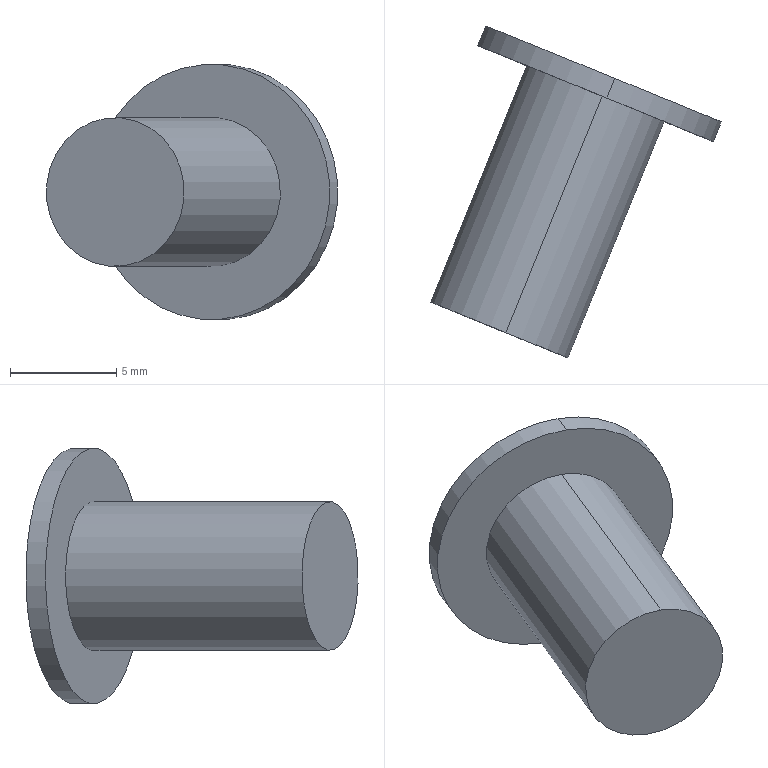Component | SolidWorks | FixedWingPin-11 | 1 solid | 7 faces | box 13.7 x 15.62 x 12 mm | volume 575 mm3 | cylinder 4 | plane 3 | commonest cylinder face diameters 12 x2 7 x2
build123d program:
from build123d import *

# Parameters (mm, degrees)
SKETCH1_R           = 3.5
BOSS_EXTRUDE1_DEPTH = 12
SKETCH2_R           = 6
BOSS_EXTRUDE2_DEPTH = 1


with BuildPart() as part:
    # Sketch1 → Boss-Extrude1 (new body)
    with BuildSketch(Plane.XY):
        with Locations((-274.486, -160)):
            Circle(SKETCH1_R)
    extrude(amount=-BOSS_EXTRUDE1_DEPTH)

    # Sketch2 → Boss-Extrude2 (add)
    with BuildSketch(Plane.XY):
        with Locations((-274.486, -160)):
            Circle(SKETCH2_R)
    extrude(amount=BOSS_EXTRUDE2_DEPTH)


solid = part.part

# Placed as in the assembly
solid = solid.moved(Location((-143.809, 26.687, -192.108), (-90, 22.15, 76.477)))
STEP:
#1=COLOUR_RGB('',0.7922,0.8196,0.9333);
#2=FILL_AREA_STYLE_COLOUR('',#1);
#3=FILL_AREA_STYLE('',(#2));
#4=SURFACE_STYLE_FILL_AREA(#3);
#5=SURFACE_SIDE_STYLE('',(#4));
#6=SURFACE_STYLE_USAGE(.BOTH.,#5);
#7=PRESENTATION_STYLE_ASSIGNMENT((#6));
#8=CARTESIAN_POINT('',(-2.336,-0.2608,4.181));
#9=VERTEX_POINT('',#8);
#10=CARTESIAN_POINT('',(-2.294,-0.2778,4.652));
#11=VERTEX_POINT('',#10);
#12=CARTESIAN_POINT('',(-2.315,-0.2693,4.417));
#13=DIRECTION('',(0.377,0.9262,0.));
#14=DIRECTION('',(-0.08843,0.036,-0.9954));
#15=AXIS2_PLACEMENT_3D('',#12,#13,#14);
#16=CIRCLE('',#15,0.2362);
#17=EDGE_CURVE('',#9,#11,#16,.T.);
#18=ORIENTED_EDGE('',*,*,#17,.F.);
#19=CARTESIAN_POINT('',(-2.351,-0.2972,4.181));
#20=VERTEX_POINT('',#19);
#21=CARTESIAN_POINT('',(-2.336,-0.2608,4.181));
#22=DIRECTION('',(-0.377,-0.9262,-0.));
#23=VECTOR('',#22,39.37);
#24=LINE('',#21,#23);
#25=EDGE_CURVE('',#9,#20,#24,.T.);
#26=ORIENTED_EDGE('',*,*,#25,.T.);
#27=CARTESIAN_POINT('',(-2.309,-0.3142,4.652));
#28=VERTEX_POINT('',#27);
#29=CARTESIAN_POINT('',(-2.33,-0.3057,4.417));
#30=DIRECTION('',(0.377,0.9262,0.));
#31=DIRECTION('',(-0.08843,0.036,-0.9954));
#32=AXIS2_PLACEMENT_3D('',#29,#30,#31);
#33=CIRCLE('',#32,0.2362);
#34=EDGE_CURVE('',#20,#28,#33,.T.);
#35=ORIENTED_EDGE('',*,*,#34,.T.);
#36=CARTESIAN_POINT('',(-2.294,-0.2778,4.652));
#37=DIRECTION('',(-0.377,-0.9262,-0.));
#38=VECTOR('',#37,39.37);
#39=LINE('',#36,#38);
#40=EDGE_CURVE('',#11,#28,#39,.T.);
#41=ORIENTED_EDGE('',*,*,#40,.F.);
#42=EDGE_LOOP('',(#18,#26,#35,#41));
#43=FACE_OUTER_BOUND('',#42,.T.);
#44=CARTESIAN_POINT('',(-2.315,-0.2693,4.417));
#45=DIRECTION('',(-0.377,-0.9262,-0.));
#46=DIRECTION('',(0.08843,-0.036,0.9954));
#47=AXIS2_PLACEMENT_3D('',#44,#45,#46);
#48=CYLINDRICAL_SURFACE('',#47,0.2362);
#49=ADVANCED_FACE('',(#43),#48,.T.);
#50=CARTESIAN_POINT('',(-2.52,-0.7384,4.279));
#51=VERTEX_POINT('',#50);
#52=CARTESIAN_POINT('',(-2.496,-0.7483,4.554));
#53=VERTEX_POINT('',#52);
#54=CARTESIAN_POINT('',(-2.508,-0.7433,4.417));
#55=DIRECTION('',(0.377,0.9262,0.));
#56=DIRECTION('',(-0.08843,0.036,-0.9954));
#57=AXIS2_PLACEMENT_3D('',#54,#55,#56);
#58=CIRCLE('',#57,0.1378);
#59=EDGE_CURVE('',#51,#53,#58,.T.);
#60=ORIENTED_EDGE('',*,*,#59,.T.);
#61=CARTESIAN_POINT('',(-2.318,-0.3107,4.554));
#62=VERTEX_POINT('',#61);
#63=CARTESIAN_POINT('',(-2.496,-0.7483,4.554));
#64=DIRECTION('',(0.377,0.9262,0.));
#65=VECTOR('',#64,39.37);
#66=LINE('',#63,#65);
#67=EDGE_CURVE('',#53,#62,#66,.T.);
#68=ORIENTED_EDGE('',*,*,#67,.T.);
#69=CARTESIAN_POINT('',(-2.342,-0.3008,4.279));
#70=VERTEX_POINT('',#69);
#71=CARTESIAN_POINT('',(-2.33,-0.3057,4.417));
#72=DIRECTION('',(0.377,0.9262,0.));
#73=DIRECTION('',(-0.08843,0.036,-0.9954));
#74=AXIS2_PLACEMENT_3D('',#71,#72,#73);
#75=CIRCLE('',#74,0.1378);
#76=EDGE_CURVE('',#70,#62,#75,.T.);
#77=ORIENTED_EDGE('',*,*,#76,.F.);
#78=CARTESIAN_POINT('',(-2.52,-0.7384,4.279));
#79=DIRECTION('',(0.377,0.9262,0.));
#80=VECTOR('',#79,39.37);
#81=LINE('',#78,#80);
#82=EDGE_CURVE('',#51,#70,#81,.T.);
#83=ORIENTED_EDGE('',*,*,#82,.F.);
#84=EDGE_LOOP('',(#60,#68,#77,#83));
#85=FACE_OUTER_BOUND('',#84,.T.);
#86=CARTESIAN_POINT('',(-2.508,-0.7433,4.417));
#87=DIRECTION('',(0.377,0.9262,0.));
#88=DIRECTION('',(-0.08843,0.036,-0.9954));
#89=AXIS2_PLACEMENT_3D('',#86,#87,#88);
#90=CYLINDRICAL_SURFACE('',#89,0.1378);
#91=ADVANCED_FACE('',(#85),#90,.T.);
#92=ORIENTED_EDGE('',*,*,#67,.F.);
#93=CARTESIAN_POINT('',(-2.508,-0.7433,4.417));
#94=DIRECTION('',(0.377,0.9262,0.));
#95=DIRECTION('',(-0.08843,0.036,-0.9954));
#96=AXIS2_PLACEMENT_3D('',#93,#94,#95);
#97=CIRCLE('',#96,0.1378);
#98=EDGE_CURVE('',#53,#51,#97,.T.);
#99=ORIENTED_EDGE('',*,*,#98,.T.);
#100=ORIENTED_EDGE('',*,*,#82,.T.);
#101=CARTESIAN_POINT('',(-2.33,-0.3057,4.417));
#102=DIRECTION('',(0.377,0.9262,0.));
#103=DIRECTION('',(-0.08843,0.036,-0.9954));
#104=AXIS2_PLACEMENT_3D('',#101,#102,#103);
#105=CIRCLE('',#104,0.1378);
#106=EDGE_CURVE('',#62,#70,#105,.T.);
#107=ORIENTED_EDGE('',*,*,#106,.F.);
#108=EDGE_LOOP('',(#92,#99,#100,#107));
#109=FACE_OUTER_BOUND('',#108,.T.);
#110=CARTESIAN_POINT('',(-2.508,-0.7433,4.417));
#111=DIRECTION('',(0.377,0.9262,0.));
#112=DIRECTION('',(-0.08843,0.036,-0.9954));
#113=AXIS2_PLACEMENT_3D('',#110,#111,#112);
#114=CYLINDRICAL_SURFACE('',#113,0.1378);
#115=ADVANCED_FACE('',(#109),#114,.T.);
#116=ORIENTED_EDGE('',*,*,#59,.F.);
#117=ORIENTED_EDGE('',*,*,#98,.F.);
#118=EDGE_LOOP('',(#116,#117));
#119=FACE_OUTER_BOUND('',#118,.T.);
#120=CARTESIAN_POINT('',(-2.508,-0.7433,4.417));
#121=DIRECTION('',(0.377,0.9262,0.));
#122=DIRECTION('',(-0.08843,0.036,-0.9954));
#123=AXIS2_PLACEMENT_3D('',#120,#121,#122);
#124=PLANE('',#123);
#125=ADVANCED_FACE('',(#119),#124,.F.);
#126=ORIENTED_EDGE('',*,*,#25,.F.);
#127=CARTESIAN_POINT('',(-2.315,-0.2693,4.417));
#128=DIRECTION('',(0.377,0.9262,0.));
#129=DIRECTION('',(-0.08843,0.036,-0.9954));
#130=AXIS2_PLACEMENT_3D('',#127,#128,#129);
#131=CIRCLE('',#130,0.2362);
#132=EDGE_CURVE('',#11,#9,#131,.T.);
#133=ORIENTED_EDGE('',*,*,#132,.F.);
#134=ORIENTED_EDGE('',*,*,#40,.T.);
#135=CARTESIAN_POINT('',(-2.33,-0.3057,4.417));
#136=DIRECTION('',(0.377,0.9262,0.));
#137=DIRECTION('',(-0.08843,0.036,-0.9954));
#138=AXIS2_PLACEMENT_3D('',#135,#136,#137);
#139=CIRCLE('',#138,0.2362);
#140=EDGE_CURVE('',#28,#20,#139,.T.);
#141=ORIENTED_EDGE('',*,*,#140,.T.);
#142=EDGE_LOOP('',(#126,#133,#134,#141));
#143=FACE_OUTER_BOUND('',#142,.T.);
#144=CARTESIAN_POINT('',(-2.315,-0.2693,4.417));
#145=DIRECTION('',(-0.377,-0.9262,-0.));
#146=DIRECTION('',(0.08843,-0.036,0.9954));
#147=AXIS2_PLACEMENT_3D('',#144,#145,#146);
#148=CYLINDRICAL_SURFACE('',#147,0.2362);
#149=ADVANCED_FACE('',(#143),#148,.T.);
#150=ORIENTED_EDGE('',*,*,#132,.T.);
#151=ORIENTED_EDGE('',*,*,#17,.T.);
#152=EDGE_LOOP('',(#150,#151));
#153=FACE_OUTER_BOUND('',#152,.T.);
#154=CARTESIAN_POINT('',(-2.315,-0.2693,4.417));
#155=DIRECTION('',(0.377,0.9262,0.));
#156=DIRECTION('',(-0.08843,0.036,-0.9954));
#157=AXIS2_PLACEMENT_3D('',#154,#155,#156);
#158=PLANE('',#157);
#159=ADVANCED_FACE('',(#153),#158,.T.);
#160=ORIENTED_EDGE('',*,*,#76,.T.);
#161=ORIENTED_EDGE('',*,*,#106,.T.);
#162=EDGE_LOOP('',(#160,#161));
#163=FACE_BOUND('',#162,.T.);
#164=ORIENTED_EDGE('',*,*,#140,.F.);
#165=ORIENTED_EDGE('',*,*,#34,.F.);
#166=EDGE_LOOP('',(#164,#165));
#167=FACE_OUTER_BOUND('',#166,.T.);
#168=CARTESIAN_POINT('',(-2.33,-0.3057,4.417));
#169=DIRECTION('',(0.377,0.9262,0.));
#170=DIRECTION('',(-0.08843,0.036,-0.9954));
#171=AXIS2_PLACEMENT_3D('',#168,#169,#170);
#172=PLANE('',#171);
#173=ADVANCED_FACE('',(#163,#167),#172,.F.);
#174=CLOSED_SHELL('',(#49,#91,#115,#125,#149,#159,#173));
#175=MANIFOLD_SOLID_BREP('',#174);
#176=STYLED_ITEM('',(#7),#175);
#177=(LENGTH_UNIT()NAMED_UNIT(*)SI_UNIT($,.METRE.));
#178=LENGTH_MEASURE_WITH_UNIT(LENGTH_MEASURE(0.0254),#177);
#179=DIMENSIONAL_EXPONENTS(1.,0.,0.,0.,0.,0.,0.);
#180=(CONVERSION_BASED_UNIT('',#178)LENGTH_UNIT()NAMED_UNIT(#179));
#181=UNCERTAINTY_MEASURE_WITH_UNIT(LENGTH_MEASURE(0.00001),#180,'','');
#182=(NAMED_UNIT(*)PLANE_ANGLE_UNIT()SI_UNIT($,.RADIAN.));
#183=(NAMED_UNIT(*)SI_UNIT($,.STERADIAN.)SOLID_ANGLE_UNIT());
#184=(GEOMETRIC_REPRESENTATION_CONTEXT(3)GLOBAL_UNCERTAINTY_ASSIGNED_CONTEXT((#181))GLOBAL_UNIT_ASSIGNED_CONTEXT((#180,#182,#183))REPRESENTATION_CONTEXT('',''));
#185=MECHANICAL_DESIGN_GEOMETRIC_PRESENTATION_REPRESENTATION('',(#176),#184);
#186=CARTESIAN_POINT('',(0.,0.,0.));
#187=DIRECTION('',(0.,0.,1.));
#188=DIRECTION('',(1.,0.,0.));
#189=AXIS2_PLACEMENT_3D('',#186,#187,#188);
#190=(LENGTH_UNIT()NAMED_UNIT(*)SI_UNIT($,.METRE.));
#191=LENGTH_MEASURE_WITH_UNIT(LENGTH_MEASURE(0.0254),#190);
#192=DIMENSIONAL_EXPONENTS(1.,0.,0.,0.,0.,0.,0.);
#193=(CONVERSION_BASED_UNIT('',#191)LENGTH_UNIT()NAMED_UNIT(#192));
#194=UNCERTAINTY_MEASURE_WITH_UNIT(LENGTH_MEASURE(0.00001),#193,'','');
#195=(NAMED_UNIT(*)PLANE_ANGLE_UNIT()SI_UNIT($,.RADIAN.));
#196=(NAMED_UNIT(*)SI_UNIT($,.STERADIAN.)SOLID_ANGLE_UNIT());
#197=(GEOMETRIC_REPRESENTATION_CONTEXT(3)GLOBAL_UNCERTAINTY_ASSIGNED_CONTEXT((#194))GLOBAL_UNIT_ASSIGNED_CONTEXT((#193,#195,#196))REPRESENTATION_CONTEXT('',''));
#198=ADVANCED_BREP_SHAPE_REPRESENTATION('',(#175,#189),#197);
#199=PRESENTATION_LAYER_ASSIGNMENT('','',(#176));